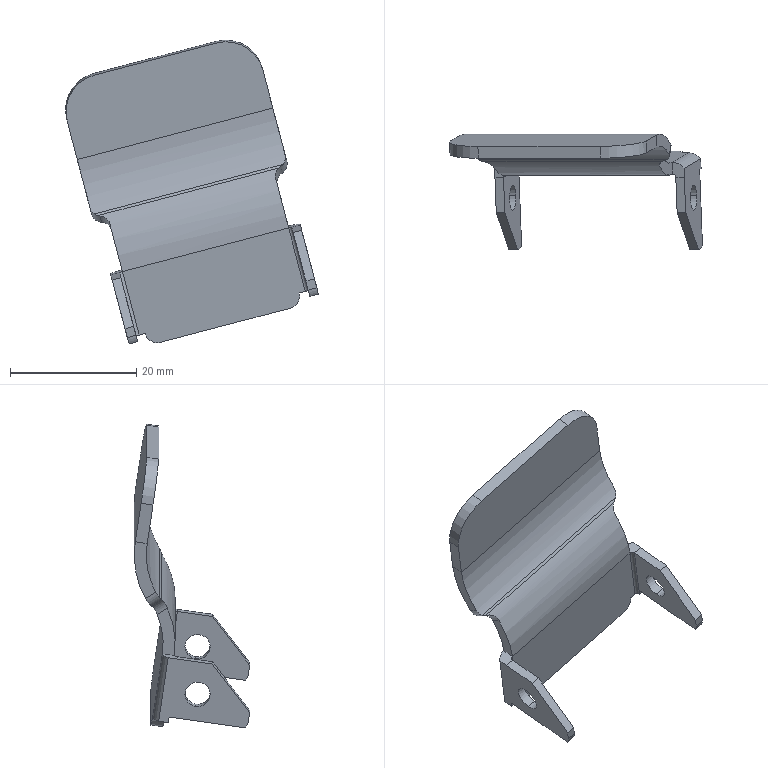Component | SolidWorks | PC-CAJ-P08-1_Rueda 2 in AZUL-1_Pieza4-1 | 1 solid | 58 faces | volume 2796 mm3 | plane 36 | cylinder 22 | commonest cylinder face diameters 4 x12 1 x2 4.8 x2 12 x2 27.8 x1 24 x1 26.2 x1 30 x1 | material Plain Carbon Steel